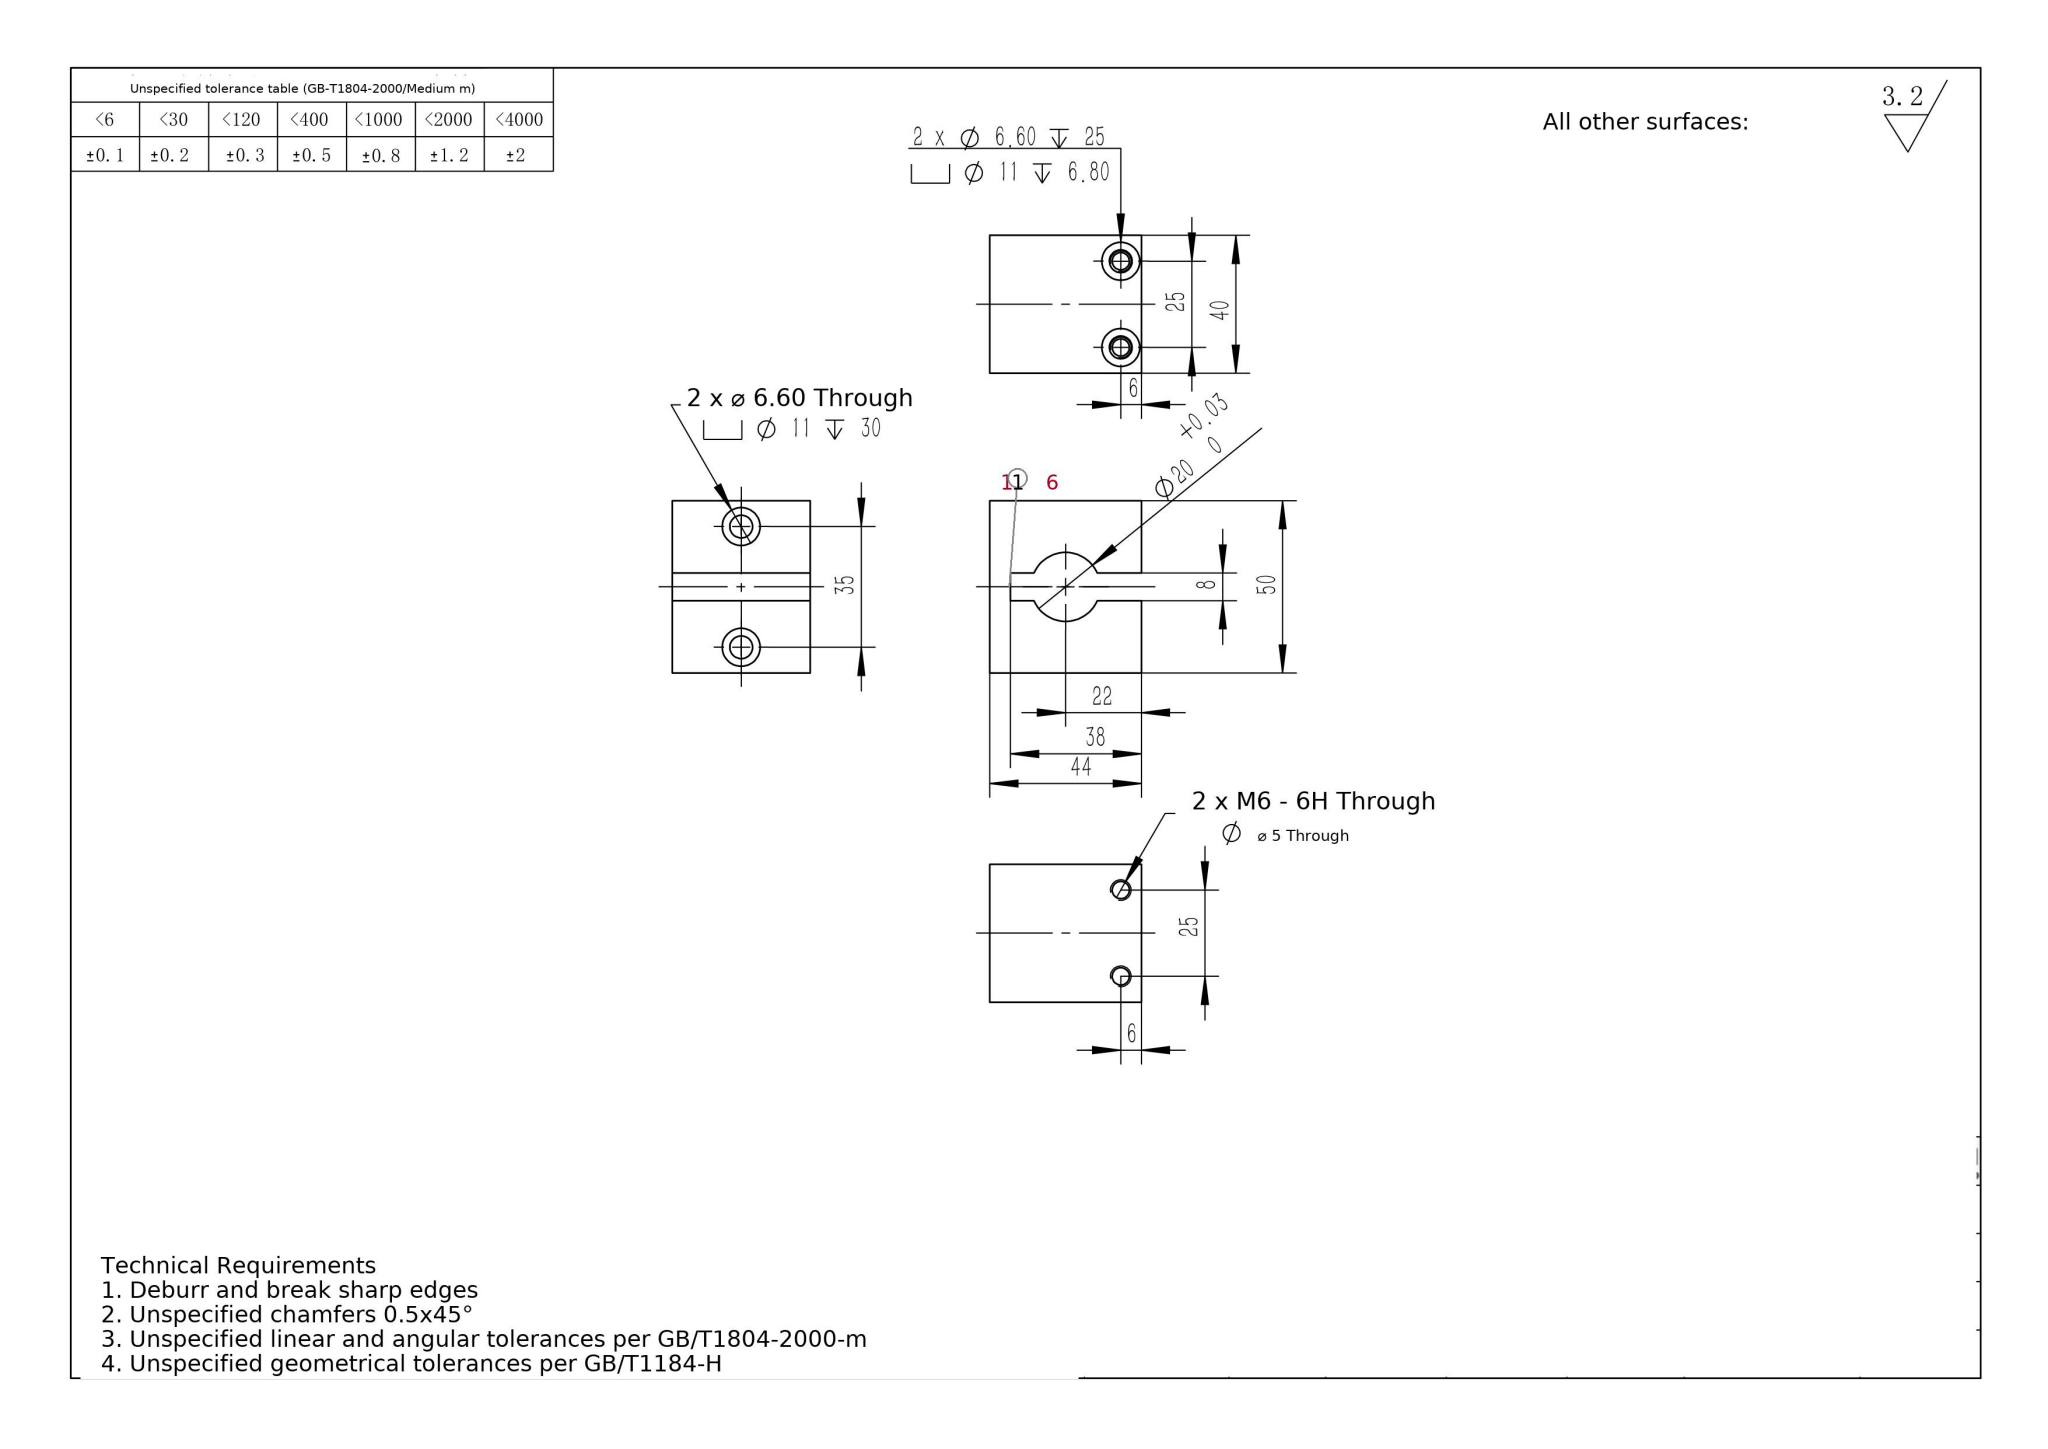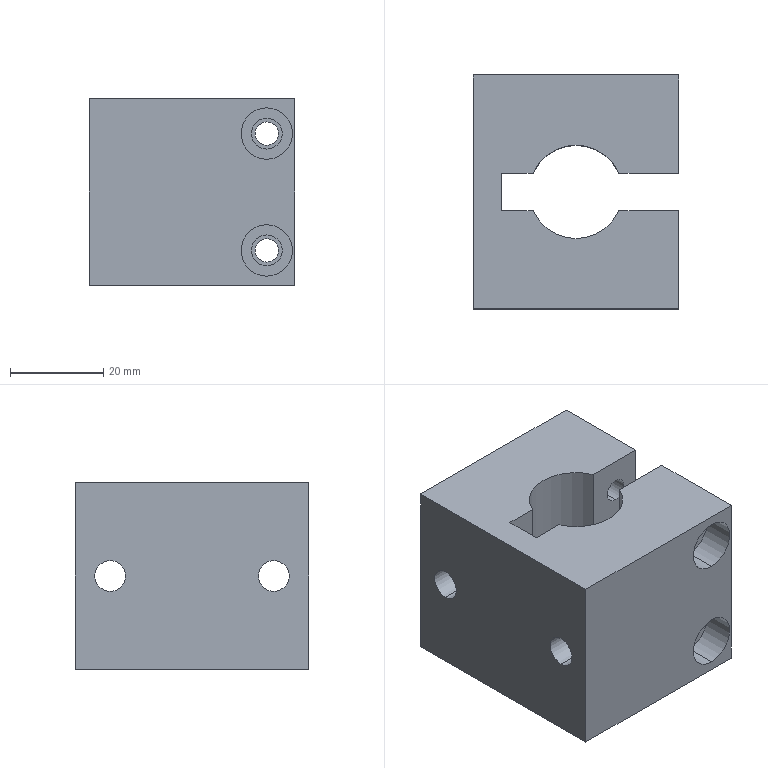Part | SolidWorks | mm | 1 solid | 38 faces | box 44 x 50 x 40 mm | volume 59750 mm3 | cylinder 22 | plane 16 | commonest cylinder face diameters 11 x8 6.6 x8 5 x4 20 x2
build123d program:
from build123d import *

# Parameters (mm, degrees)
BOSS_EXTRUDE1_DEPTH                               = 40
HOLE_SIZE_ACCORDING_TO_TYPE_2_OF_HEXA_D           = 6.6
HOLE_SIZE_ACCORDING_TO_TYPE_2_OF_HEXA_CBORE_D     = 11
HOLE_SIZE_ACCORDING_TO_TYPE_2_OF_HEXA_CBORE_DEPTH = 30
HOLE_SIZE_ACCORDING_TO_TYPE_2_OF_2_D              = 6.6
HOLE_SIZE_ACCORDING_TO_TYPE_2_OF_2_DEPTH          = 25
HOLE_SIZE_ACCORDING_TO_TYPE_2_OF_2_CBORE_D        = 11
HOLE_SIZE_ACCORDING_TO_TYPE_2_OF_2_CBORE_DEPTH    = 6.8
HOLE_SIZE_ACCORDING_TO_TYPE_2_OF_2_TIP            = 1.983
M6_TAPPED_HOLE1_D                                 = 5


with BuildPart() as part:
    # Sketch1 → Boss-Extrude1 (new body)
    with BuildSketch(Plane.XY):
        with BuildLine():
            Line((0, 25), (0, -25))
            Line((0, -25), (44, -25))
            Line((44, -25), (44, -4))
            Line((44, -4), (31.165, -4))
            ThreePointArc((31.165, -4), (22, -10), (12.835, -4))
            Line((12.835, -4), (6, -4))
            Line((6, -4), (6, 4))
            Line((6, 4), (12.835, 4))
            ThreePointArc((12.835, 4), (22, 10), (31.165, 4))
            Line((31.165, 4), (44, 4))
            Line((44, 4), (44, 25))
            Line((44, 25), (0, 25))
        make_face()
    extrude(amount=BOSS_EXTRUDE1_DEPTH)

    # Hole Size _ according to_ Type 2 of Hexa (through all)
    with Locations(Plane(origin=(44, 0, 0), x_dir=(0, 0, -1), z_dir=(1, 0, 0))):
        with Locations((-20, 17.5), (-20, -17.5)):
            CounterBoreHole(HOLE_SIZE_ACCORDING_TO_TYPE_2_OF_HEXA_D / 2, HOLE_SIZE_ACCORDING_TO_TYPE_2_OF_HEXA_CBORE_D / 2, HOLE_SIZE_ACCORDING_TO_TYPE_2_OF_HEXA_CBORE_DEPTH)

    # Hole Size _ according to_ Type 2 of  2
    with Locations(Plane(origin=(0, -25, 0), x_dir=(-1, 0, 0), z_dir=(0, -1, 0))):
        with Locations((-38, -32.5), (-38, -7.5)):
            CounterBoreHole(HOLE_SIZE_ACCORDING_TO_TYPE_2_OF_2_D / 2, HOLE_SIZE_ACCORDING_TO_TYPE_2_OF_2_CBORE_D / 2, HOLE_SIZE_ACCORDING_TO_TYPE_2_OF_2_CBORE_DEPTH, depth=HOLE_SIZE_ACCORDING_TO_TYPE_2_OF_2_DEPTH)
            with Locations((0, 0, -(HOLE_SIZE_ACCORDING_TO_TYPE_2_OF_2_DEPTH + HOLE_SIZE_ACCORDING_TO_TYPE_2_OF_2_TIP / 2))):  # 118° drill point
                Cone(0, HOLE_SIZE_ACCORDING_TO_TYPE_2_OF_2_D / 2, HOLE_SIZE_ACCORDING_TO_TYPE_2_OF_2_TIP, mode=Mode.SUBTRACT)

    # M6 Tapped Hole1 (through all)
    with Locations(Plane(origin=(0, 4, 0), x_dir=(-1, 0, 0), z_dir=(0, -1, 0))):
        with Locations((-38, -32.5), (-38, -7.5)):
            Hole(M6_TAPPED_HOLE1_D / 2)


solid = part.part